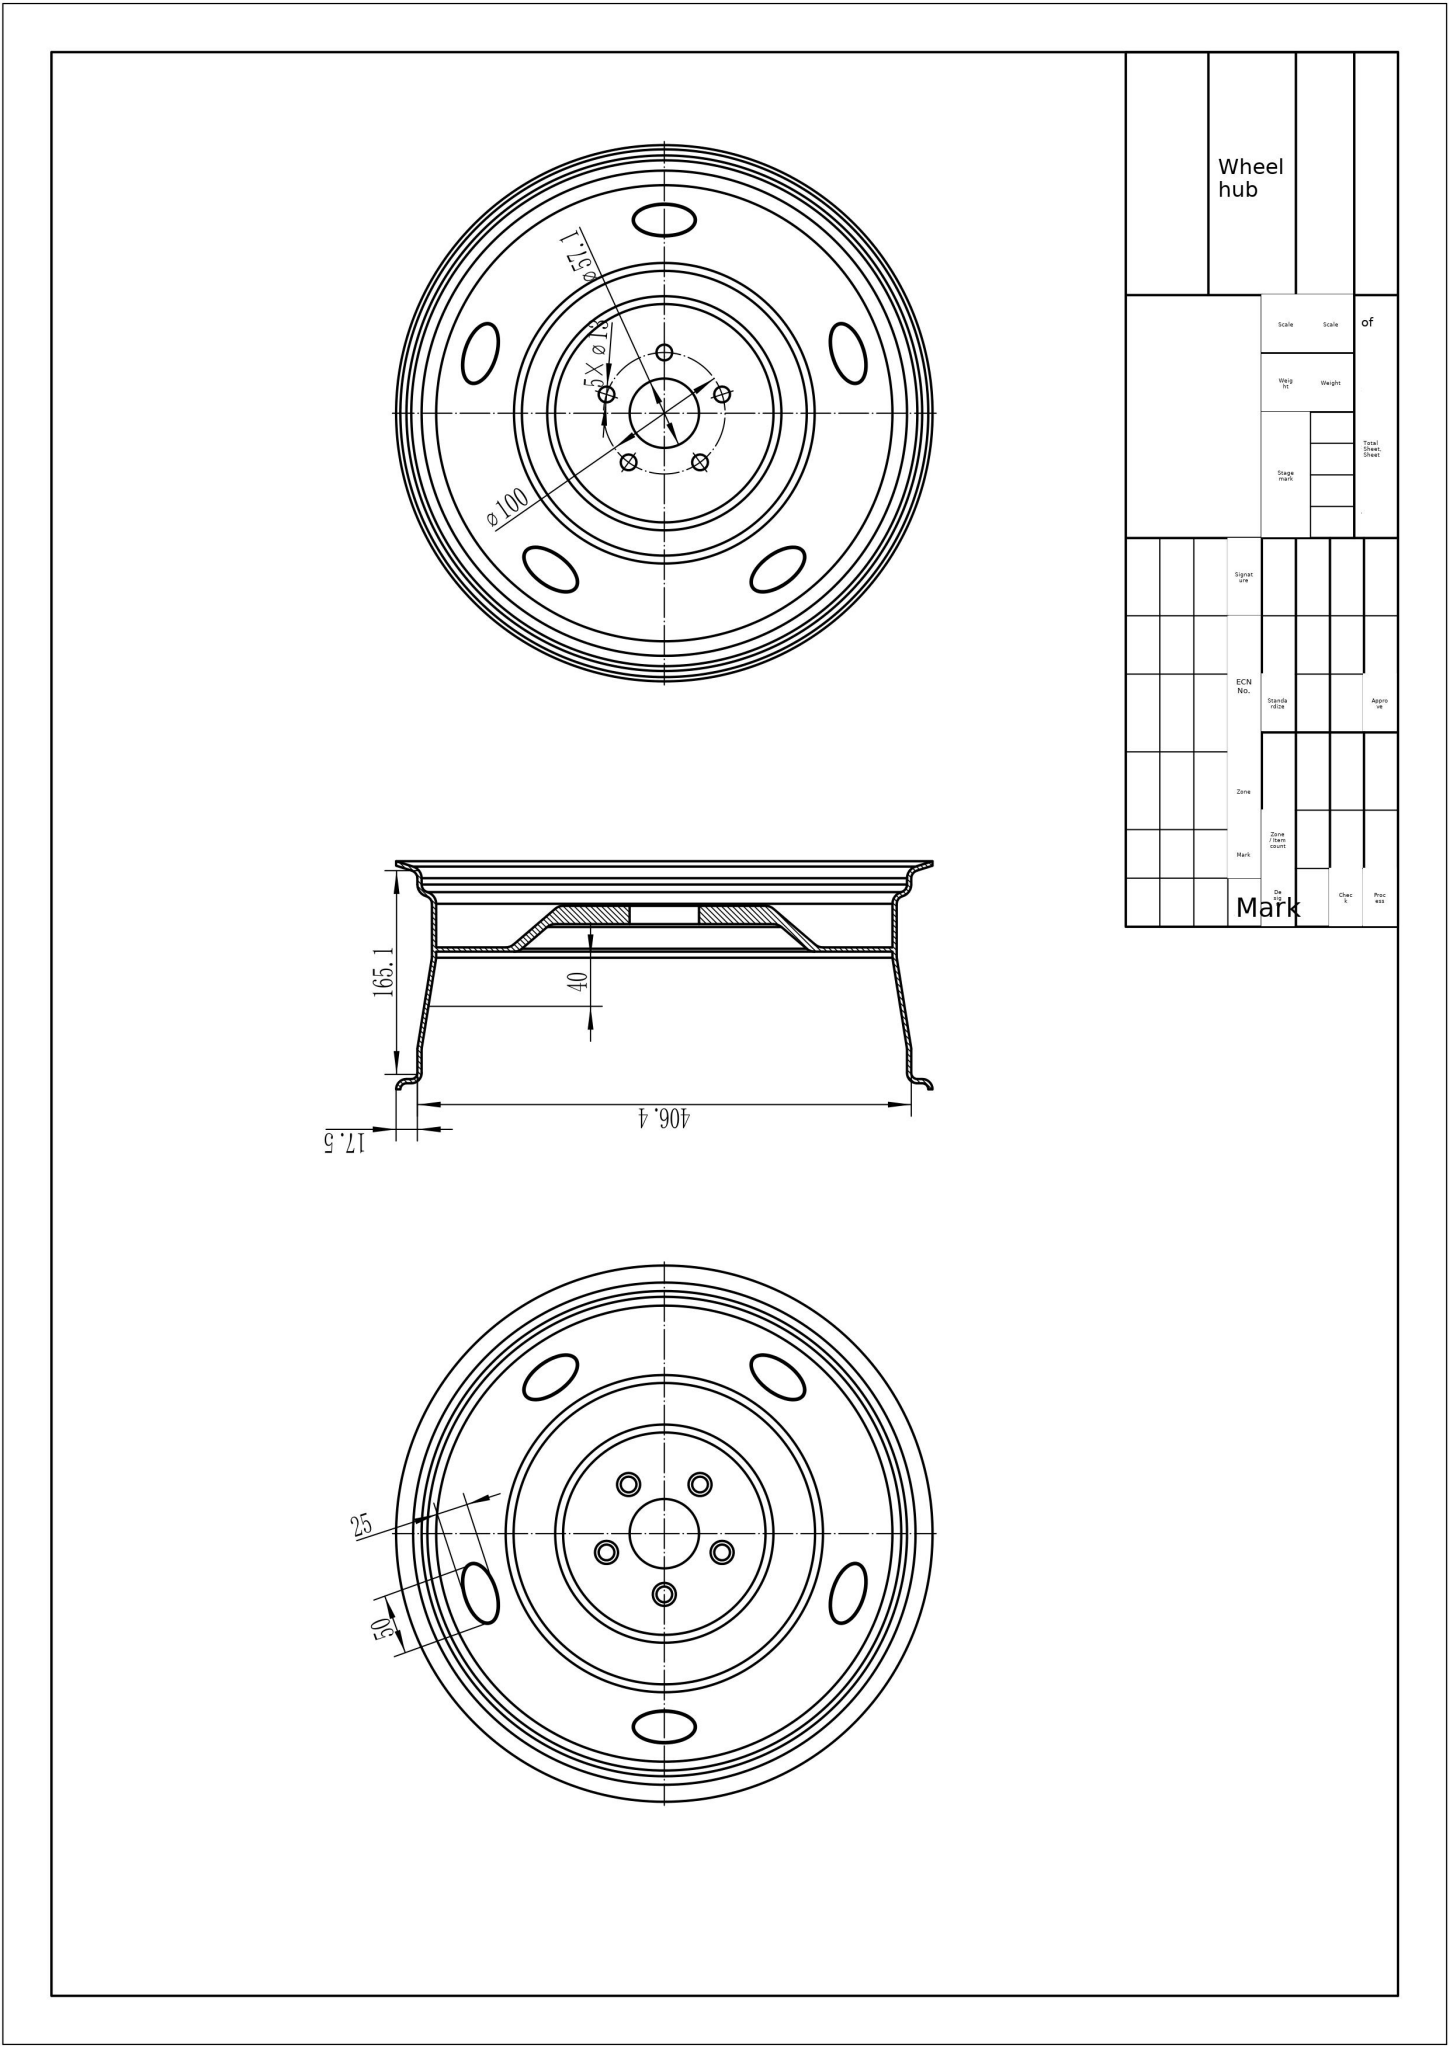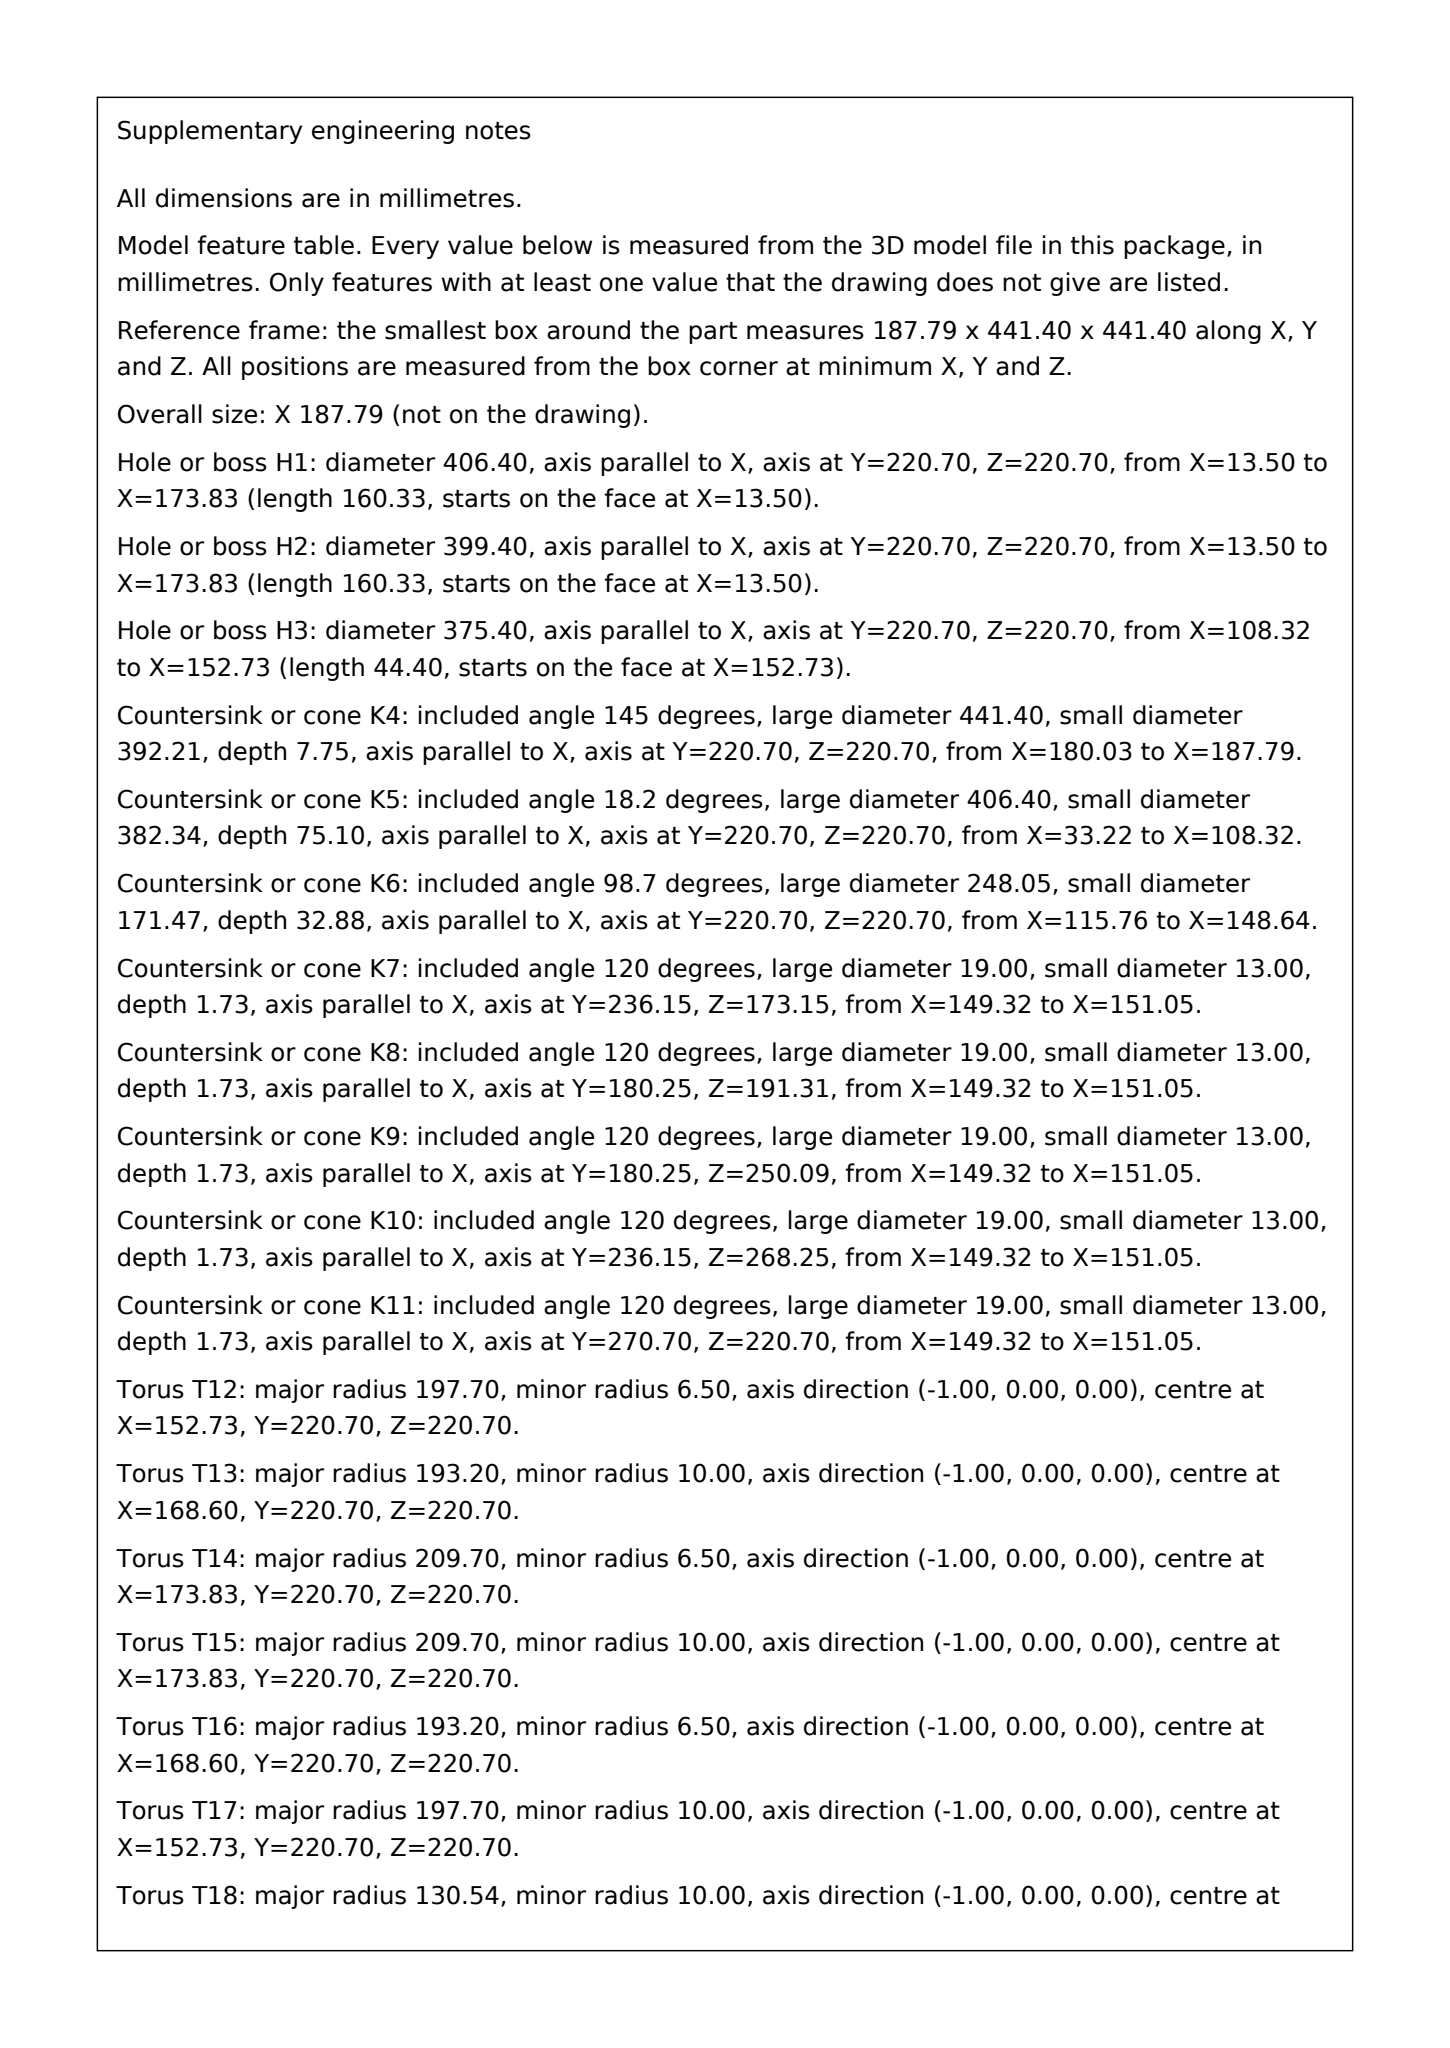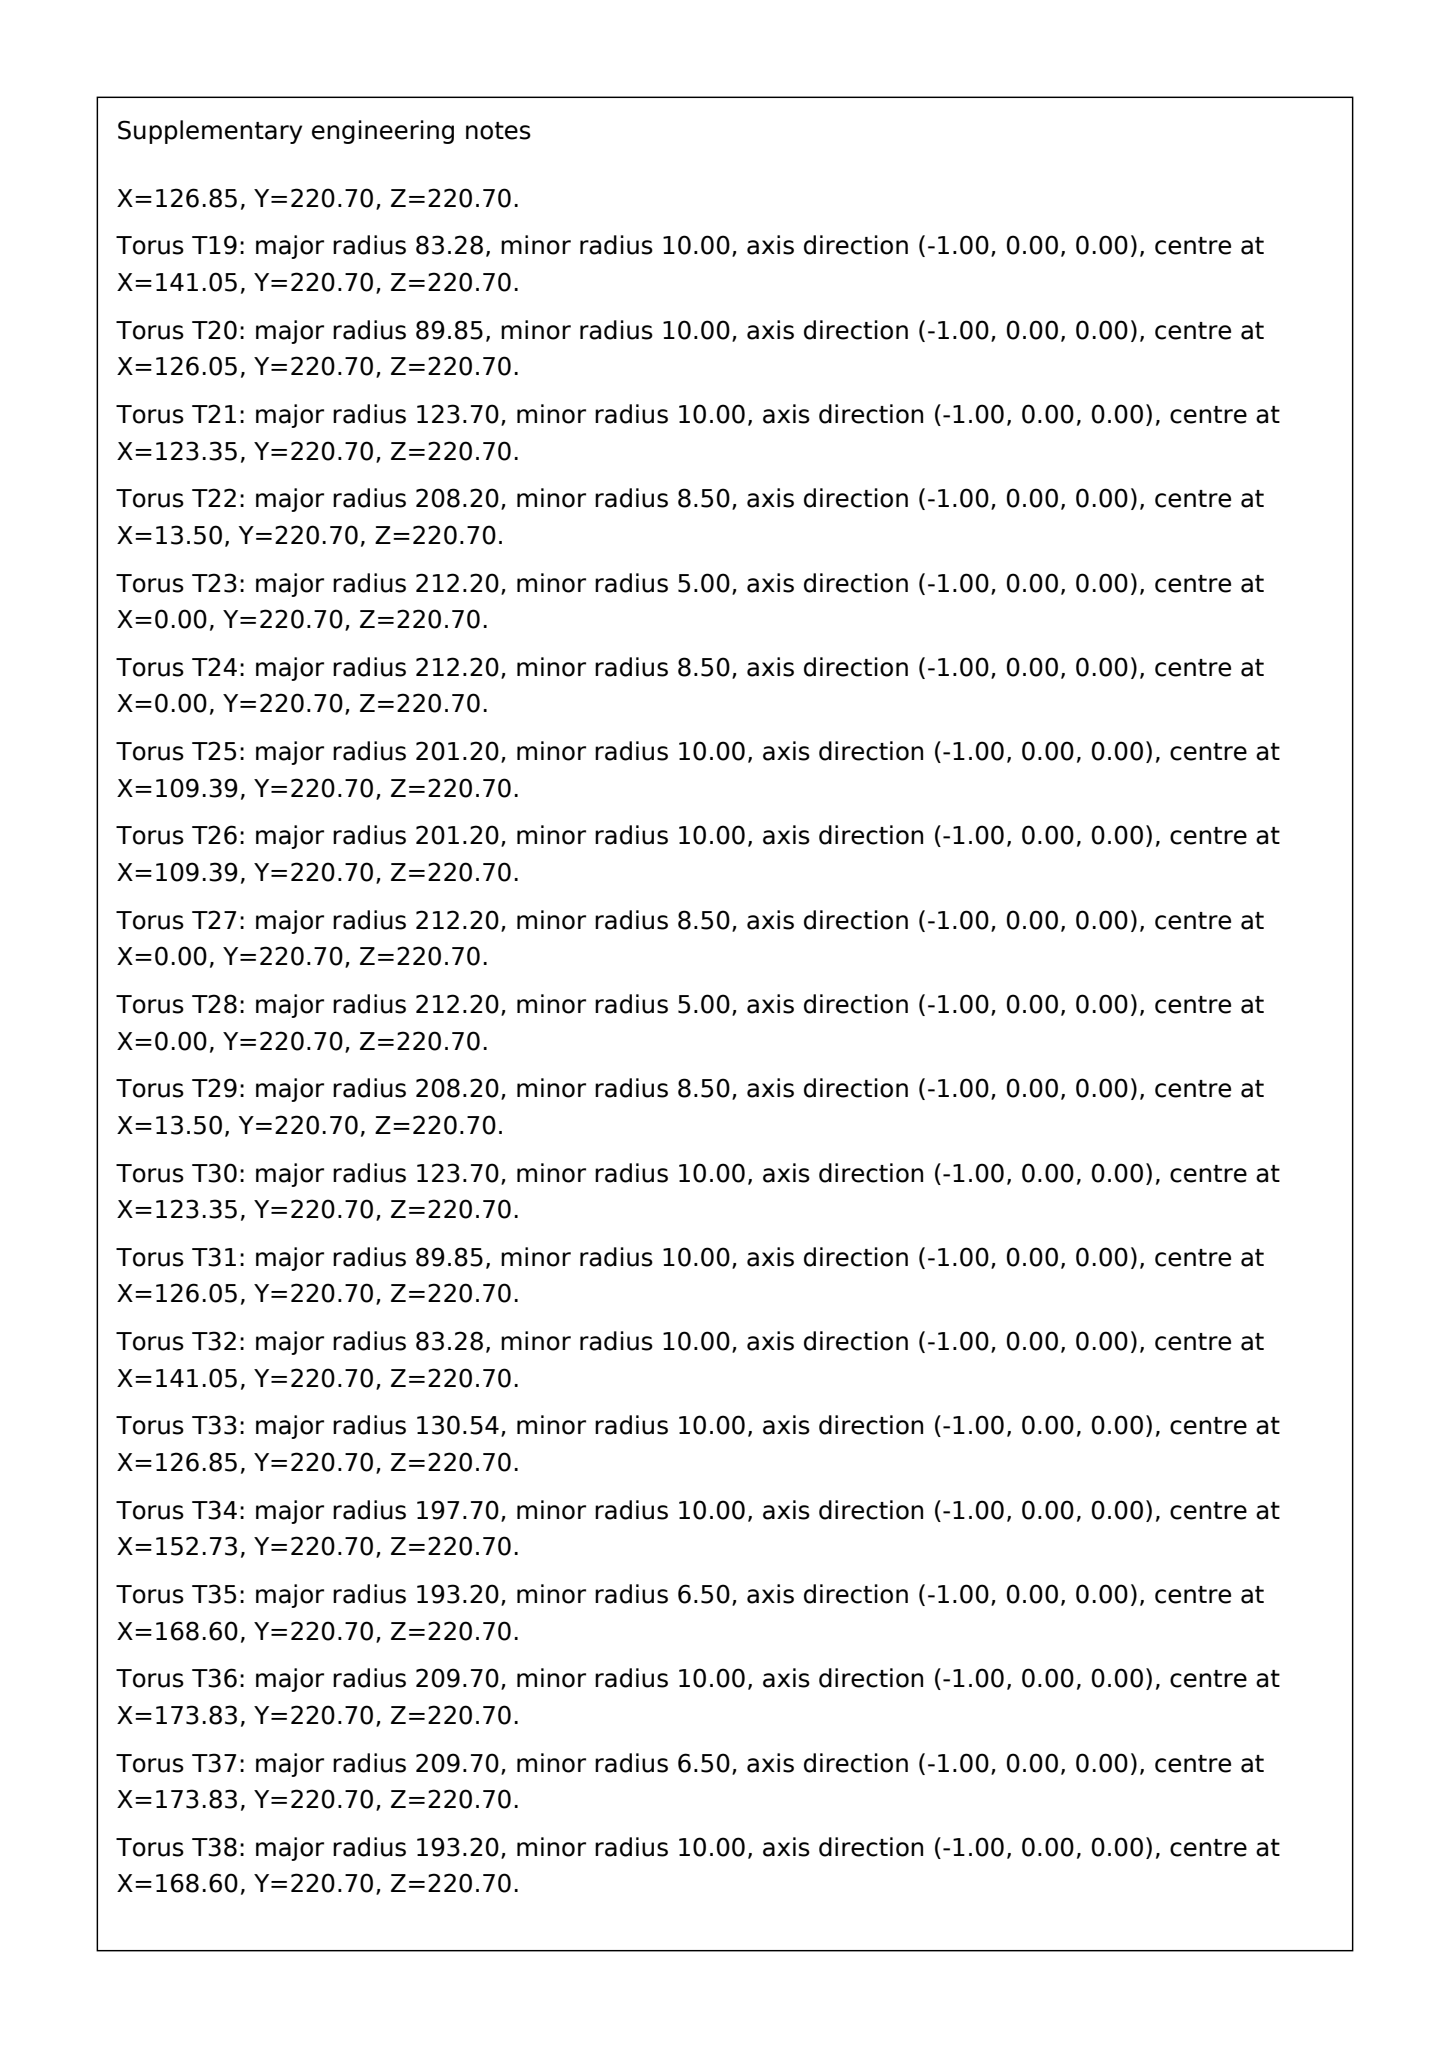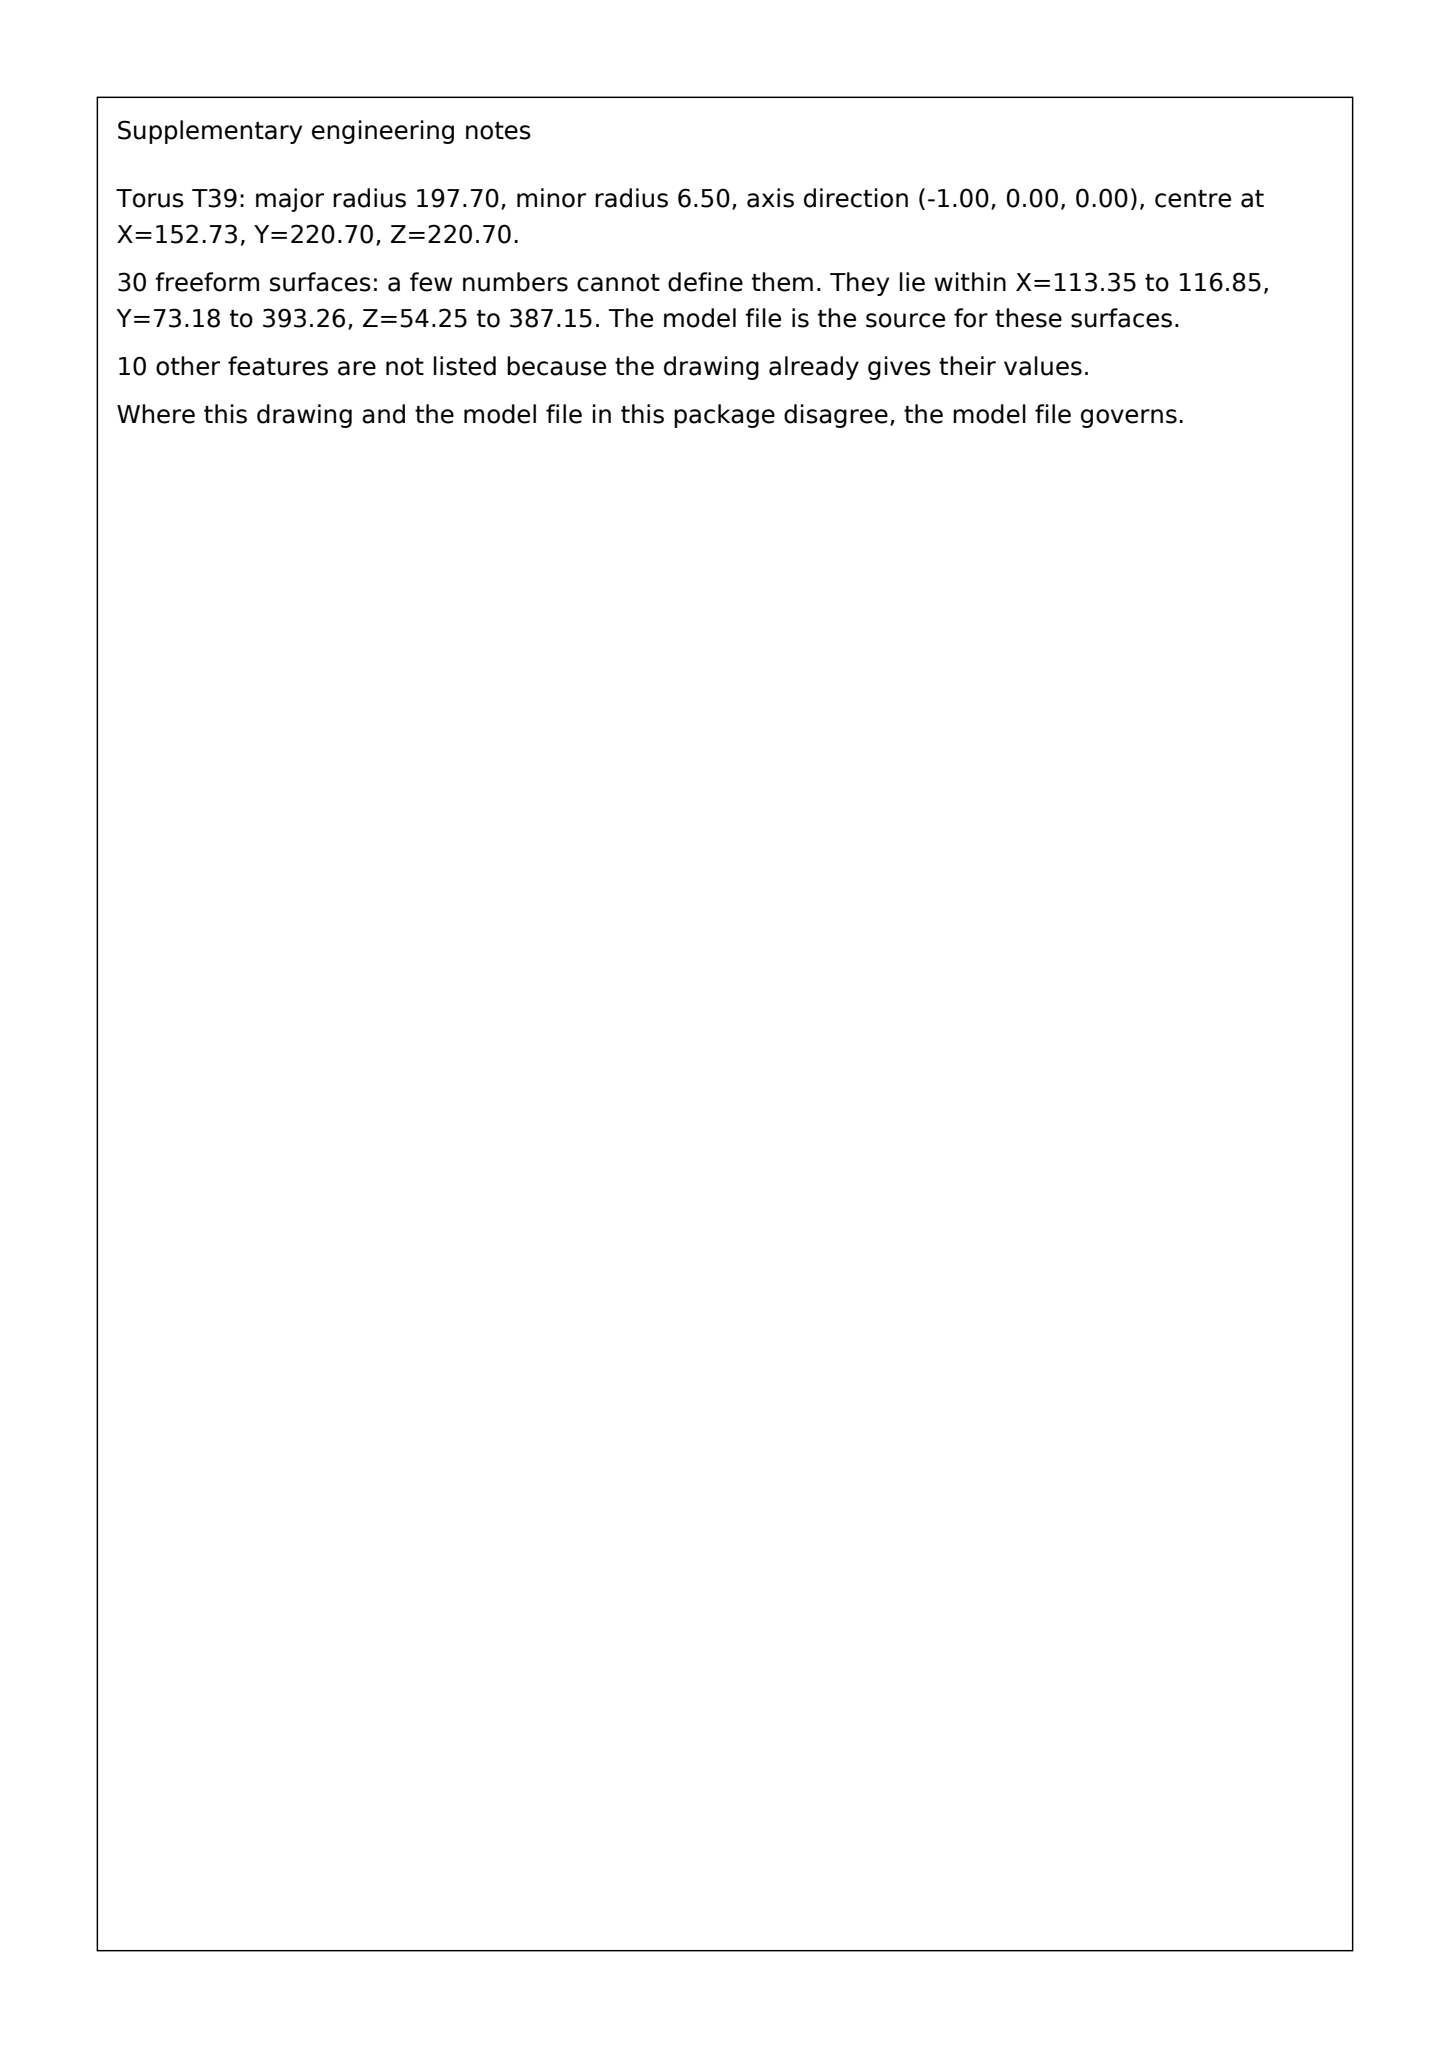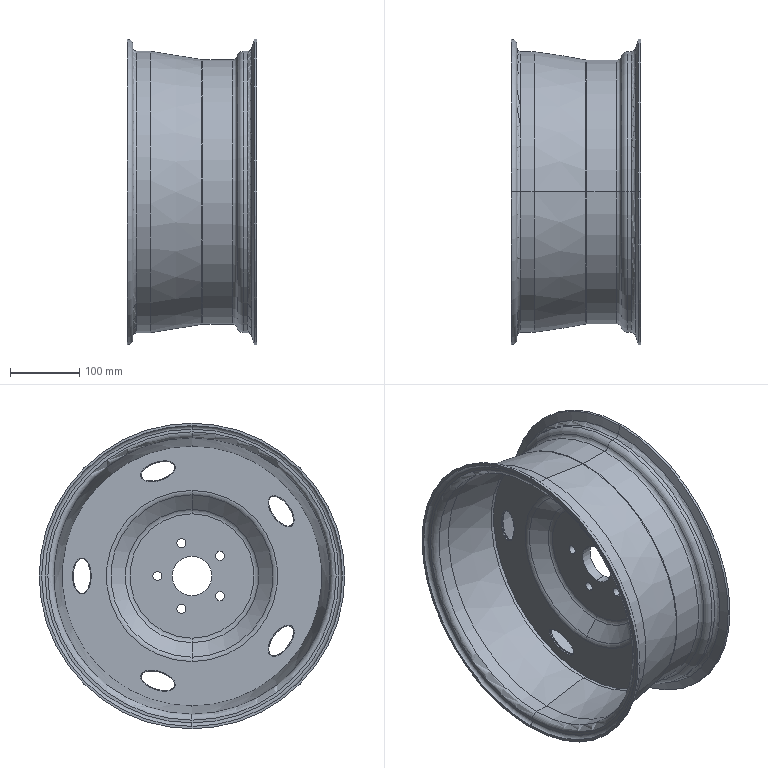Part | SolidWorks | mm | 1 solid | 117 faces | box 187.79 x 441.4 x 441.4 mm | volume 1690177 mm3 | spline 30 | torus 30 | cylinder 28 | cone 22 | plane 7 | commonest cylinder face diameters 13 x10 406.4 x4 399.4 x4 375.4 x4 382.4 x2 441.4 x2 57.1 x2
build123d program:
from build123d import *

# Parameters (mm, degrees)
SKETCH2_R          = 6.5
CUT_EXTRUDE1_DEPTH = 347.746
CHAMFER1_SIZE      = 3
CHAMFER1_SIZE2     = 1.732
SKETCH3_RX         = 25
SKETCH3_RY         = 12.5
CUT_EXTRUDE2_DEPTH = 10
FILLET1_R          = 1


with BuildPart() as part:
    # Sketch1 → Revolve3 (revolve)
    with BuildSketch(Plane.XY, mode=Mode.PRIVATE) as revolve3_sk:
        with BuildLine():
            Line((40, 89.847), (40, 28.55))
            Line((40, 28.55), (55, 28.55))
            Line((55, 28.55), (55, 83.282))
            ThreePointArc((55, 83.282), (54.378, 86.754), (52.589, 89.795))
            Line((52.589, 89.795), (23.213, 124.026))
            ThreePointArc((23.213, 124.026), (21.424, 127.066), (20.801, 130.538))
            Line((20.801, 130.538), (20.801, 187.7))
            Line((20.801, 187.7), (56.675, 187.7))
            ThreePointArc((56.675, 187.7), (62.706, 189.723), (66.296, 194.973))
            ThreePointArc((66.296, 194.973), (68.63, 198.385), (72.55, 199.7))
            Line((72.55, 199.7), (77.784, 199.7))
            ThreePointArc((77.784, 199.7), (83.697, 201.636), (87.321, 206.693))
            Line((87.321, 206.693), (91.738, 220.7))
            Line((91.738, 220.7), (88.068, 220.7))
            Line((88.068, 220.7), (83.983, 207.745))
            ThreePointArc((83.983, 207.745), (81.628, 204.458), (77.784, 203.2))
            Line((77.784, 203.2), (72.55, 203.2))
            ThreePointArc((72.55, 203.2), (66.52, 201.177), (62.929, 195.927))
            ThreePointArc((62.929, 195.927), (60.595, 192.515), (56.675, 191.2))
            Line((56.675, 191.2), (13.344, 191.2))
            ThreePointArc((13.344, 191.2), (12.552, 191.231), (11.766, 191.325))
            Line((11.766, 191.325), (-62.55, 203.2))
            Line((-62.55, 203.2), (-82.55, 203.2))
            ThreePointArc((-82.55, 203.2), (-86.086, 204.664), (-87.55, 208.2))
            Line((-87.55, 208.2), (-87.55, 212.2))
            ThreePointArc((-87.55, 212.2), (-90.04, 218.21), (-96.05, 220.7))
            Line((-96.05, 220.7), (-96.05, 217.2))
            ThreePointArc((-96.05, 217.2), (-92.514, 215.736), (-91.05, 212.2))
            Line((-91.05, 212.2), (-91.05, 208.2))
            ThreePointArc((-91.05, 208.2), (-88.56, 202.19), (-82.55, 199.7))
            Line((-82.55, 199.7), (-62.828, 199.7))
            Line((-62.828, 199.7), (12.272, 187.7))
            Line((12.272, 187.7), (17.301, 187.7))
            Line((17.301, 187.7), (17.301, 123.703))
            ThreePointArc((17.301, 123.703), (17.924, 120.23), (19.713, 117.19))
            Line((19.713, 117.19), (37.589, 96.36))
            ThreePointArc((37.589, 96.36), (39.378, 93.32), (40, 89.847))
        make_face()
    revolve(revolve3_sk.sketch.rotate(Axis((-158.518, 0, 0), (1, 0, 0)), 90), axis=Axis((-158.518, 0, 0), (1, 0, 0)))

    # Sketch2 → Cut-Extrude1 (cut, through all)
    with BuildSketch(Plane(origin=(55, 0, 0), x_dir=(0, 0, -1), z_dir=(1, 0, 0))):
        with Locations((0, 50)):
            Circle(SKETCH2_R)
        with Locations((47.553, 15.451)):
            Circle(SKETCH2_R)
        with Locations((29.389, -40.451)):
            Circle(SKETCH2_R)
        with Locations((-29.389, -40.451)):
            Circle(SKETCH2_R)
        with Locations((-47.553, 15.451)):
            Circle(SKETCH2_R)
    extrude(amount=-CUT_EXTRUDE1_DEPTH, mode=Mode.SUBTRACT)

    # Chamfer1
    chamfer1_edges = [part.edges().sort_by_distance(p)[0] for p in [
        (55, 15.451, 54.053),
        (55, 50, 6.5),
        (55, 15.451, -41.053),
        (55, -40.451, -22.889),
        (55, -40.451, 35.889),
    ]]
    chamfer1_side = [part.faces().sort_by_distance(p)[0] for p in [
        (55, 0, -80.927),
    ]]
    chamfer(chamfer1_edges, length=CHAMFER1_SIZE, length2=CHAMFER1_SIZE2, reference=chamfer1_side[0])

    # Sketch3 → Cut-Extrude2 (cut)
    with BuildSketch(Plane(origin=(20.801, 0, 0), x_dir=(0, 0, -1), z_dir=(1, 0, 0))):
        with Locations(Location((0, 159.058), (0, 0, 0))):
            Ellipse(SKETCH3_RX, SKETCH3_RY)
        with Locations(Location((151.273, 49.152), (0, 0, -72))):
            Ellipse(SKETCH3_RX, SKETCH3_RY)
        with Locations(Location((93.492, -128.68), (0, 0, -144))):
            Ellipse(SKETCH3_RX, SKETCH3_RY)
        with Locations(Location((-93.492, -128.68), (0, 0, -36))):
            Ellipse(SKETCH3_RX, SKETCH3_RY)
        with Locations(Location((-151.273, 49.152), (0, 0, 72))):
            Ellipse(SKETCH3_RX, SKETCH3_RY)
    extrude(amount=-CUT_EXTRUDE2_DEPTH, mode=Mode.SUBTRACT)

    # Fillet1
    fillet1_edges = [part.edges().sort_by_distance(p)[0] for p in [
        (17.301, 159.058, 25),
        (20.801, 158.978, 24.999),
        (17.301, 72.928, -143.548),
        (20.801, 72.903, -143.472),
        (17.301, -113.986, -113.717),
        (20.801, -113.922, -113.67),
        (17.301, -113.986, 113.717),
        (20.801, -114.05, 113.764),
        (17.301, 25.375, 158.998),
        (20.801, 25.351, 158.923),
    ]]
    fillet(fillet1_edges, radius=FILLET1_R)


solid = part.part